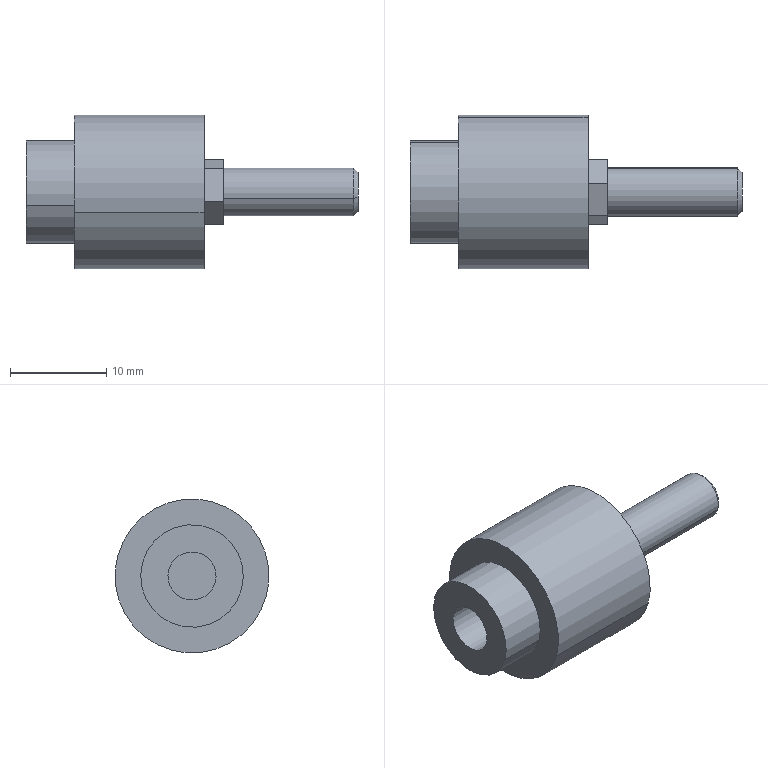Component | SolidWorks | JA15_5_080-2 | 1 solid | 22 faces | box 34.5 x 16 x 16 mm | volume 3290 mm3 | plane 12 | cylinder 8 | cone 2 | commonest cylinder face diameters 5 x4 10.667 x2 16 x2 | material 45
STEP:
#1=COLOUR_RGB('',0.7922,0.8196,0.9333);
#2=FILL_AREA_STYLE_COLOUR('',#1);
#3=FILL_AREA_STYLE('',(#2));
#4=SURFACE_STYLE_FILL_AREA(#3);
#5=SURFACE_SIDE_STYLE('',(#4));
#6=SURFACE_STYLE_USAGE(.BOTH.,#5);
#7=PRESENTATION_STYLE_ASSIGNMENT((#6));
#8=CARTESIAN_POINT('',(4.538,0.8016,3.156));
#9=VERTEX_POINT('',#8);
#10=CARTESIAN_POINT('',(4.538,0.9912,3.209));
#11=VERTEX_POINT('',#10);
#12=CARTESIAN_POINT('',(4.538,0.8964,3.182));
#13=DIRECTION('',(-1.,-0.,-0.));
#14=DIRECTION('',(0.,0.9628,0.2701));
#15=AXIS2_PLACEMENT_3D('',#12,#13,#14);
#16=CIRCLE('',#15,0.09843);
#17=EDGE_CURVE('',#9,#11,#16,.T.);
#18=ORIENTED_EDGE('',*,*,#17,.T.);
#19=CARTESIAN_POINT('',(4.952,0.9912,3.209));
#20=VERTEX_POINT('',#19);
#21=CARTESIAN_POINT('',(4.125,0.9912,3.209));
#22=DIRECTION('',(1.,0.,0.));
#23=VECTOR('',#22,39.37);
#24=LINE('',#21,#23);
#25=EDGE_CURVE('',#11,#20,#24,.T.);
#26=ORIENTED_EDGE('',*,*,#25,.T.);
#27=CARTESIAN_POINT('',(4.952,0.8016,3.156));
#28=VERTEX_POINT('',#27);
#29=CARTESIAN_POINT('',(4.952,0.8964,3.182));
#30=DIRECTION('',(1.,0.,0.));
#31=DIRECTION('',(0.,-0.9628,-0.2701));
#32=AXIS2_PLACEMENT_3D('',#29,#30,#31);
#33=CIRCLE('',#32,0.09843);
#34=EDGE_CURVE('',#20,#28,#33,.T.);
#35=ORIENTED_EDGE('',*,*,#34,.T.);
#36=CARTESIAN_POINT('',(4.125,0.8016,3.156));
#37=DIRECTION('',(1.,0.,0.));
#38=VECTOR('',#37,39.37);
#39=LINE('',#36,#38);
#40=EDGE_CURVE('',#9,#28,#39,.T.);
#41=ORIENTED_EDGE('',*,*,#40,.F.);
#42=EDGE_LOOP('',(#18,#26,#35,#41));
#43=FACE_OUTER_BOUND('',#42,.T.);
#44=CARTESIAN_POINT('',(4.125,0.8964,3.182));
#45=DIRECTION('',(1.,0.,0.));
#46=DIRECTION('',(0.,-0.9628,-0.2701));
#47=AXIS2_PLACEMENT_3D('',#44,#45,#46);
#48=CYLINDRICAL_SURFACE('',#47,0.09843);
#49=ADVANCED_FACE('',(#43),#48,.F.);
#50=CARTESIAN_POINT('',(5.877,0.9912,3.209));
#51=VERTEX_POINT('',#50);
#52=CARTESIAN_POINT('',(5.877,0.8016,3.156));
#53=VERTEX_POINT('',#52);
#54=CARTESIAN_POINT('',(5.877,0.8964,3.182));
#55=DIRECTION('',(-1.,-0.,-0.));
#56=DIRECTION('',(0.,0.9628,0.2701));
#57=AXIS2_PLACEMENT_3D('',#54,#55,#56);
#58=CIRCLE('',#57,0.09843);
#59=EDGE_CURVE('',#51,#53,#58,.T.);
#60=ORIENTED_EDGE('',*,*,#59,.T.);
#61=CARTESIAN_POINT('',(5.345,0.8016,3.156));
#62=VERTEX_POINT('',#61);
#63=CARTESIAN_POINT('',(5.345,0.8016,3.156));
#64=DIRECTION('',(-1.,-0.,-0.));
#65=VECTOR('',#64,39.37);
#66=LINE('',#63,#65);
#67=EDGE_CURVE('',#53,#62,#66,.T.);
#68=ORIENTED_EDGE('',*,*,#67,.T.);
#69=CARTESIAN_POINT('',(5.345,0.9912,3.209));
#70=VERTEX_POINT('',#69);
#71=CARTESIAN_POINT('',(5.345,0.8964,3.182));
#72=DIRECTION('',(1.,0.,0.));
#73=DIRECTION('',(0.,-0.9628,-0.2701));
#74=AXIS2_PLACEMENT_3D('',#71,#72,#73);
#75=CIRCLE('',#74,0.09843);
#76=EDGE_CURVE('',#62,#70,#75,.T.);
#77=ORIENTED_EDGE('',*,*,#76,.T.);
#78=CARTESIAN_POINT('',(5.345,0.9912,3.209));
#79=DIRECTION('',(-1.,-0.,-0.));
#80=VECTOR('',#79,39.37);
#81=LINE('',#78,#80);
#82=EDGE_CURVE('',#51,#70,#81,.T.);
#83=ORIENTED_EDGE('',*,*,#82,.F.);
#84=EDGE_LOOP('',(#60,#68,#77,#83));
#85=FACE_OUTER_BOUND('',#84,.T.);
#86=CARTESIAN_POINT('',(5.345,0.8964,3.182));
#87=DIRECTION('',(-1.,-0.,-0.));
#88=DIRECTION('',(0.,0.9628,0.2701));
#89=AXIS2_PLACEMENT_3D('',#86,#87,#88);
#90=CYLINDRICAL_SURFACE('',#89,0.09843);
#91=ADVANCED_FACE('',(#85),#90,.T.);
#92=CARTESIAN_POINT('',(5.896,0.9726,3.204));
#93=VERTEX_POINT('',#92);
#94=CARTESIAN_POINT('',(5.896,0.8202,3.161));
#95=VERTEX_POINT('',#94);
#96=CARTESIAN_POINT('',(5.896,0.8964,3.182));
#97=DIRECTION('',(-1.,-0.,-0.));
#98=DIRECTION('',(0.,0.9628,0.2701));
#99=AXIS2_PLACEMENT_3D('',#96,#97,#98);
#100=CIRCLE('',#99,0.07913);
#101=EDGE_CURVE('',#93,#95,#100,.T.);
#102=ORIENTED_EDGE('',*,*,#101,.T.);
#103=CARTESIAN_POINT('',(5.877,0.8016,3.156));
#104=DIRECTION('',(-0.7071,-0.6808,-0.191));
#105=VECTOR('',#104,39.37);
#106=LINE('',#103,#105);
#107=EDGE_CURVE('',#95,#53,#106,.T.);
#108=ORIENTED_EDGE('',*,*,#107,.T.);
#109=ORIENTED_EDGE('',*,*,#59,.F.);
#110=CARTESIAN_POINT('',(5.877,0.9912,3.209));
#111=DIRECTION('',(-0.7071,0.6808,0.191));
#112=VECTOR('',#111,39.37);
#113=LINE('',#110,#112);
#114=EDGE_CURVE('',#93,#51,#113,.T.);
#115=ORIENTED_EDGE('',*,*,#114,.F.);
#116=EDGE_LOOP('',(#102,#108,#109,#115));
#117=FACE_OUTER_BOUND('',#116,.T.);
#118=CARTESIAN_POINT('',(5.877,0.8964,3.182));
#119=DIRECTION('',(-1.,-0.,-0.));
#120=DIRECTION('',(0.,0.9628,0.2701));
#121=AXIS2_PLACEMENT_3D('',#118,#119,#120);
#122=CONICAL_SURFACE('',#121,0.09843,0.7854);
#123=ADVANCED_FACE('',(#117),#122,.T.);
#124=CARTESIAN_POINT('',(4.735,1.099,3.239));
#125=VERTEX_POINT('',#124);
#126=CARTESIAN_POINT('',(4.735,0.6942,3.126));
#127=VERTEX_POINT('',#126);
#128=CARTESIAN_POINT('',(4.735,0.8964,3.182));
#129=DIRECTION('',(-1.,-0.,-0.));
#130=DIRECTION('',(0.,0.9628,0.2701));
#131=AXIS2_PLACEMENT_3D('',#128,#129,#130);
#132=CIRCLE('',#131,0.21);
#133=EDGE_CURVE('',#125,#127,#132,.T.);
#134=ORIENTED_EDGE('',*,*,#133,.T.);
#135=CARTESIAN_POINT('',(4.538,0.6942,3.126));
#136=VERTEX_POINT('',#135);
#137=CARTESIAN_POINT('',(4.538,0.6942,3.126));
#138=DIRECTION('',(-1.,-0.,-0.));
#139=VECTOR('',#138,39.37);
#140=LINE('',#137,#139);
#141=EDGE_CURVE('',#127,#136,#140,.T.);
#142=ORIENTED_EDGE('',*,*,#141,.T.);
#143=CARTESIAN_POINT('',(4.538,1.099,3.239));
#144=VERTEX_POINT('',#143);
#145=CARTESIAN_POINT('',(4.538,0.8964,3.182));
#146=DIRECTION('',(-1.,-0.,-0.));
#147=DIRECTION('',(0.,0.9628,0.2701));
#148=AXIS2_PLACEMENT_3D('',#145,#146,#147);
#149=CIRCLE('',#148,0.21);
#150=EDGE_CURVE('',#144,#136,#149,.T.);
#151=ORIENTED_EDGE('',*,*,#150,.F.);
#152=CARTESIAN_POINT('',(4.538,1.099,3.239));
#153=DIRECTION('',(-1.,-0.,-0.));
#154=VECTOR('',#153,39.37);
#155=LINE('',#152,#154);
#156=EDGE_CURVE('',#125,#144,#155,.T.);
#157=ORIENTED_EDGE('',*,*,#156,.F.);
#158=EDGE_LOOP('',(#134,#142,#151,#157));
#159=FACE_OUTER_BOUND('',#158,.T.);
#160=CARTESIAN_POINT('',(4.538,0.8964,3.182));
#161=DIRECTION('',(-1.,-0.,-0.));
#162=DIRECTION('',(0.,0.9628,0.2701));
#163=AXIS2_PLACEMENT_3D('',#160,#161,#162);
#164=CYLINDRICAL_SURFACE('',#163,0.21);
#165=ADVANCED_FACE('',(#159),#164,.T.);
#166=CARTESIAN_POINT('',(5.267,1.2,3.267));
#167=VERTEX_POINT('',#166);
#168=CARTESIAN_POINT('',(5.267,0.5931,3.097));
#169=VERTEX_POINT('',#168);
#170=CARTESIAN_POINT('',(5.267,0.8964,3.182));
#171=DIRECTION('',(-1.,-0.,-0.));
#172=DIRECTION('',(0.,0.9628,0.2701));
#173=AXIS2_PLACEMENT_3D('',#170,#171,#172);
#174=CIRCLE('',#173,0.315);
#175=EDGE_CURVE('',#167,#169,#174,.T.);
#176=ORIENTED_EDGE('',*,*,#175,.T.);
#177=CARTESIAN_POINT('',(4.735,0.5931,3.097));
#178=VERTEX_POINT('',#177);
#179=CARTESIAN_POINT('',(4.538,0.5931,3.097));
#180=DIRECTION('',(-1.,-0.,-0.));
#181=VECTOR('',#180,39.37);
#182=LINE('',#179,#181);
#183=EDGE_CURVE('',#169,#178,#182,.T.);
#184=ORIENTED_EDGE('',*,*,#183,.T.);
#185=CARTESIAN_POINT('',(4.735,1.2,3.267));
#186=VERTEX_POINT('',#185);
#187=CARTESIAN_POINT('',(4.735,0.8964,3.182));
#188=DIRECTION('',(-1.,-0.,-0.));
#189=DIRECTION('',(0.,0.9628,0.2701));
#190=AXIS2_PLACEMENT_3D('',#187,#188,#189);
#191=CIRCLE('',#190,0.315);
#192=EDGE_CURVE('',#186,#178,#191,.T.);
#193=ORIENTED_EDGE('',*,*,#192,.F.);
#194=CARTESIAN_POINT('',(4.538,1.2,3.267));
#195=DIRECTION('',(-1.,-0.,-0.));
#196=VECTOR('',#195,39.37);
#197=LINE('',#194,#196);
#198=EDGE_CURVE('',#167,#186,#197,.T.);
#199=ORIENTED_EDGE('',*,*,#198,.F.);
#200=EDGE_LOOP('',(#176,#184,#193,#199));
#201=FACE_OUTER_BOUND('',#200,.T.);
#202=CARTESIAN_POINT('',(4.538,0.8964,3.182));
#203=DIRECTION('',(-1.,-0.,-0.));
#204=DIRECTION('',(0.,0.9628,0.2701));
#205=AXIS2_PLACEMENT_3D('',#202,#203,#204);
#206=CYLINDRICAL_SURFACE('',#205,0.315);
#207=ADVANCED_FACE('',(#201),#206,.T.);
#208=ORIENTED_EDGE('',*,*,#175,.F.);
#209=CARTESIAN_POINT('',(5.267,0.8964,3.182));
#210=DIRECTION('',(-1.,-0.,-0.));
#211=DIRECTION('',(0.,0.9628,0.2701));
#212=AXIS2_PLACEMENT_3D('',#209,#210,#211);
#213=CIRCLE('',#212,0.315);
#214=EDGE_CURVE('',#169,#167,#213,.T.);
#215=ORIENTED_EDGE('',*,*,#214,.F.);
#216=EDGE_LOOP('',(#208,#215));
#217=FACE_OUTER_BOUND('',#216,.T.);
#218=CARTESIAN_POINT('',(5.267,0.9301,3.314));
#219=VERTEX_POINT('',#218);
#220=CARTESIAN_POINT('',(5.267,0.7988,3.278));
#221=VERTEX_POINT('',#220);
#222=CARTESIAN_POINT('',(5.267,0.9301,3.314));
#223=DIRECTION('',(0.,-0.9628,-0.2701));
#224=VECTOR('',#223,39.37);
#225=LINE('',#222,#224);
#226=EDGE_CURVE('',#219,#221,#225,.T.);
#227=ORIENTED_EDGE('',*,*,#226,.F.);
#228=CARTESIAN_POINT('',(5.267,1.028,3.219));
#229=VERTEX_POINT('',#228);
#230=CARTESIAN_POINT('',(5.267,1.028,3.219));
#231=DIRECTION('',(-0.,-0.7154,0.6988));
#232=VECTOR('',#231,39.37);
#233=LINE('',#230,#232);
#234=EDGE_CURVE('',#229,#219,#233,.T.);
#235=ORIENTED_EDGE('',*,*,#234,.F.);
#236=CARTESIAN_POINT('',(5.267,0.994,3.087));
#237=VERTEX_POINT('',#236);
#238=CARTESIAN_POINT('',(5.267,0.994,3.087));
#239=DIRECTION('',(-0.,0.2475,0.9689));
#240=VECTOR('',#239,39.37);
#241=LINE('',#238,#240);
#242=EDGE_CURVE('',#237,#229,#241,.T.);
#243=ORIENTED_EDGE('',*,*,#242,.F.);
#244=CARTESIAN_POINT('',(5.267,0.8626,3.05));
#245=VERTEX_POINT('',#244);
#246=CARTESIAN_POINT('',(5.267,0.8626,3.05));
#247=DIRECTION('',(-0.,0.9628,0.2701));
#248=VECTOR('',#247,39.37);
#249=LINE('',#246,#248);
#250=EDGE_CURVE('',#245,#237,#249,.T.);
#251=ORIENTED_EDGE('',*,*,#250,.F.);
#252=CARTESIAN_POINT('',(5.267,0.7651,3.145));
#253=VERTEX_POINT('',#252);
#254=CARTESIAN_POINT('',(5.267,0.7651,3.145));
#255=DIRECTION('',(0.,0.7154,-0.6988));
#256=VECTOR('',#255,39.37);
#257=LINE('',#254,#256);
#258=EDGE_CURVE('',#253,#245,#257,.T.);
#259=ORIENTED_EDGE('',*,*,#258,.F.);
#260=CARTESIAN_POINT('',(5.267,0.7988,3.278));
#261=DIRECTION('',(0.,-0.2475,-0.9689));
#262=VECTOR('',#261,39.37);
#263=LINE('',#260,#262);
#264=EDGE_CURVE('',#221,#253,#263,.T.);
#265=ORIENTED_EDGE('',*,*,#264,.F.);
#266=EDGE_LOOP('',(#227,#235,#243,#251,#259,#265));
#267=FACE_BOUND('',#266,.T.);
#268=CARTESIAN_POINT('',(5.267,0.8964,3.182));
#269=DIRECTION('',(1.,0.,0.));
#270=DIRECTION('',(0.,-0.9628,-0.2701));
#271=AXIS2_PLACEMENT_3D('',#268,#269,#270);
#272=PLANE('',#271);
#273=ADVANCED_FACE('',(#217,#267),#272,.T.);
#274=ORIENTED_EDGE('',*,*,#183,.F.);
#275=ORIENTED_EDGE('',*,*,#214,.T.);
#276=ORIENTED_EDGE('',*,*,#198,.T.);
#277=CARTESIAN_POINT('',(4.735,0.8964,3.182));
#278=DIRECTION('',(-1.,-0.,-0.));
#279=DIRECTION('',(0.,0.9628,0.2701));
#280=AXIS2_PLACEMENT_3D('',#277,#278,#279);
#281=CIRCLE('',#280,0.315);
#282=EDGE_CURVE('',#178,#186,#281,.T.);
#283=ORIENTED_EDGE('',*,*,#282,.F.);
#284=EDGE_LOOP('',(#274,#275,#276,#283));
#285=FACE_OUTER_BOUND('',#284,.T.);
#286=CARTESIAN_POINT('',(4.538,0.8964,3.182));
#287=DIRECTION('',(-1.,-0.,-0.));
#288=DIRECTION('',(0.,0.9628,0.2701));
#289=AXIS2_PLACEMENT_3D('',#286,#287,#288);
#290=CYLINDRICAL_SURFACE('',#289,0.315);
#291=ADVANCED_FACE('',(#285),#290,.T.);
#292=ORIENTED_EDGE('',*,*,#192,.T.);
#293=ORIENTED_EDGE('',*,*,#282,.T.);
#294=EDGE_LOOP('',(#292,#293));
#295=FACE_OUTER_BOUND('',#294,.T.);
#296=ORIENTED_EDGE('',*,*,#133,.F.);
#297=CARTESIAN_POINT('',(4.735,0.8964,3.182));
#298=DIRECTION('',(-1.,-0.,-0.));
#299=DIRECTION('',(0.,0.9628,0.2701));
#300=AXIS2_PLACEMENT_3D('',#297,#298,#299);
#301=CIRCLE('',#300,0.21);
#302=EDGE_CURVE('',#127,#125,#301,.T.);
#303=ORIENTED_EDGE('',*,*,#302,.F.);
#304=EDGE_LOOP('',(#296,#303));
#305=FACE_BOUND('',#304,.T.);
#306=CARTESIAN_POINT('',(4.735,0.9815,2.879));
#307=DIRECTION('',(-1.,-0.,-0.));
#308=DIRECTION('',(-0.,0.9628,0.2701));
#309=AXIS2_PLACEMENT_3D('',#306,#307,#308);
#310=PLANE('',#309);
#311=ADVANCED_FACE('',(#295,#305),#310,.T.);
#312=ORIENTED_EDGE('',*,*,#141,.F.);
#313=ORIENTED_EDGE('',*,*,#302,.T.);
#314=ORIENTED_EDGE('',*,*,#156,.T.);
#315=CARTESIAN_POINT('',(4.538,0.8964,3.182));
#316=DIRECTION('',(-1.,-0.,-0.));
#317=DIRECTION('',(0.,0.9628,0.2701));
#318=AXIS2_PLACEMENT_3D('',#315,#316,#317);
#319=CIRCLE('',#318,0.21);
#320=EDGE_CURVE('',#136,#144,#319,.T.);
#321=ORIENTED_EDGE('',*,*,#320,.F.);
#322=EDGE_LOOP('',(#312,#313,#314,#321));
#323=FACE_OUTER_BOUND('',#322,.T.);
#324=CARTESIAN_POINT('',(4.538,0.8964,3.182));
#325=DIRECTION('',(-1.,-0.,-0.));
#326=DIRECTION('',(0.,0.9628,0.2701));
#327=AXIS2_PLACEMENT_3D('',#324,#325,#326);
#328=CYLINDRICAL_SURFACE('',#327,0.21);
#329=ADVANCED_FACE('',(#323),#328,.T.);
#330=ORIENTED_EDGE('',*,*,#150,.T.);
#331=ORIENTED_EDGE('',*,*,#320,.T.);
#332=EDGE_LOOP('',(#330,#331));
#333=FACE_OUTER_BOUND('',#332,.T.);
#334=ORIENTED_EDGE('',*,*,#17,.F.);
#335=CARTESIAN_POINT('',(4.538,0.8964,3.182));
#336=DIRECTION('',(-1.,-0.,-0.));
#337=DIRECTION('',(0.,0.9628,0.2701));
#338=AXIS2_PLACEMENT_3D('',#335,#336,#337);
#339=CIRCLE('',#338,0.09843);
#340=EDGE_CURVE('',#11,#9,#339,.T.);
#341=ORIENTED_EDGE('',*,*,#340,.F.);
#342=EDGE_LOOP('',(#334,#341));
#343=FACE_BOUND('',#342,.T.);
#344=CARTESIAN_POINT('',(4.538,0.9531,2.98));
#345=DIRECTION('',(-1.,-0.,-0.));
#346=DIRECTION('',(-0.,0.9628,0.2701));
#347=AXIS2_PLACEMENT_3D('',#344,#345,#346);
#348=PLANE('',#347);
#349=ADVANCED_FACE('',(#333,#343),#348,.T.);
#350=ORIENTED_EDGE('',*,*,#234,.T.);
#351=CARTESIAN_POINT('',(5.345,0.9301,3.314));
#352=VERTEX_POINT('',#351);
#353=CARTESIAN_POINT('',(5.345,0.9301,3.314));
#354=DIRECTION('',(-1.,-0.,-0.));
#355=VECTOR('',#354,39.37);
#356=LINE('',#353,#355);
#357=EDGE_CURVE('',#352,#219,#356,.T.);
#358=ORIENTED_EDGE('',*,*,#357,.F.);
#359=CARTESIAN_POINT('',(5.345,1.028,3.219));
#360=VERTEX_POINT('',#359);
#361=CARTESIAN_POINT('',(5.345,1.028,3.219));
#362=DIRECTION('',(-0.,-0.7154,0.6988));
#363=VECTOR('',#362,39.37);
#364=LINE('',#361,#363);
#365=EDGE_CURVE('',#360,#352,#364,.T.);
#366=ORIENTED_EDGE('',*,*,#365,.F.);
#367=CARTESIAN_POINT('',(5.345,1.028,3.219));
#368=DIRECTION('',(-1.,-0.,-0.));
#369=VECTOR('',#368,39.37);
#370=LINE('',#367,#369);
#371=EDGE_CURVE('',#360,#229,#370,.T.);
#372=ORIENTED_EDGE('',*,*,#371,.T.);
#373=EDGE_LOOP('',(#350,#358,#366,#372));
#374=FACE_OUTER_BOUND('',#373,.T.);
#375=CARTESIAN_POINT('',(5.345,1.028,3.219));
#376=DIRECTION('',(0.,-0.6988,-0.7154));
#377=DIRECTION('',(0.,0.7154,-0.6988));
#378=AXIS2_PLACEMENT_3D('',#375,#376,#377);
#379=PLANE('',#378);
#380=ADVANCED_FACE('',(#374),#379,.F.);
#381=ORIENTED_EDGE('',*,*,#226,.T.);
#382=CARTESIAN_POINT('',(5.345,0.7988,3.278));
#383=VERTEX_POINT('',#382);
#384=CARTESIAN_POINT('',(5.345,0.7988,3.278));
#385=DIRECTION('',(-1.,-0.,-0.));
#386=VECTOR('',#385,39.37);
#387=LINE('',#384,#386);
#388=EDGE_CURVE('',#383,#221,#387,.T.);
#389=ORIENTED_EDGE('',*,*,#388,.F.);
#390=CARTESIAN_POINT('',(5.345,0.9301,3.314));
#391=DIRECTION('',(0.,-0.9628,-0.2701));
#392=VECTOR('',#391,39.37);
#393=LINE('',#390,#392);
#394=EDGE_CURVE('',#352,#383,#393,.T.);
#395=ORIENTED_EDGE('',*,*,#394,.F.);
#396=ORIENTED_EDGE('',*,*,#357,.T.);
#397=EDGE_LOOP('',(#381,#389,#395,#396));
#398=FACE_OUTER_BOUND('',#397,.T.);
#399=CARTESIAN_POINT('',(5.345,0.9301,3.314));
#400=DIRECTION('',(0.,0.2701,-0.9628));
#401=DIRECTION('',(1.,0.,0.));
#402=AXIS2_PLACEMENT_3D('',#399,#400,#401);
#403=PLANE('',#402);
#404=ADVANCED_FACE('',(#398),#403,.F.);
#405=ORIENTED_EDGE('',*,*,#264,.T.);
#406=CARTESIAN_POINT('',(5.345,0.7651,3.145));
#407=VERTEX_POINT('',#406);
#408=CARTESIAN_POINT('',(5.345,0.7651,3.145));
#409=DIRECTION('',(-1.,-0.,-0.));
#410=VECTOR('',#409,39.37);
#411=LINE('',#408,#410);
#412=EDGE_CURVE('',#407,#253,#411,.T.);
#413=ORIENTED_EDGE('',*,*,#412,.F.);
#414=CARTESIAN_POINT('',(5.345,0.7988,3.278));
#415=DIRECTION('',(0.,-0.2475,-0.9689));
#416=VECTOR('',#415,39.37);
#417=LINE('',#414,#416);
#418=EDGE_CURVE('',#383,#407,#417,.T.);
#419=ORIENTED_EDGE('',*,*,#418,.F.);
#420=ORIENTED_EDGE('',*,*,#388,.T.);
#421=EDGE_LOOP('',(#405,#413,#419,#420));
#422=FACE_OUTER_BOUND('',#421,.T.);
#423=CARTESIAN_POINT('',(5.345,0.7988,3.278));
#424=DIRECTION('',(0.,0.9689,-0.2475));
#425=DIRECTION('',(-0.,0.2475,0.9689));
#426=AXIS2_PLACEMENT_3D('',#423,#424,#425);
#427=PLANE('',#426);
#428=ADVANCED_FACE('',(#422),#427,.F.);
#429=ORIENTED_EDGE('',*,*,#258,.T.);
#430=CARTESIAN_POINT('',(5.345,0.8626,3.05));
#431=VERTEX_POINT('',#430);
#432=CARTESIAN_POINT('',(5.345,0.8626,3.05));
#433=DIRECTION('',(-1.,-0.,-0.));
#434=VECTOR('',#433,39.37);
#435=LINE('',#432,#434);
#436=EDGE_CURVE('',#431,#245,#435,.T.);
#437=ORIENTED_EDGE('',*,*,#436,.F.);
#438=CARTESIAN_POINT('',(5.345,0.7651,3.145));
#439=DIRECTION('',(0.,0.7154,-0.6988));
#440=VECTOR('',#439,39.37);
#441=LINE('',#438,#440);
#442=EDGE_CURVE('',#407,#431,#441,.T.);
#443=ORIENTED_EDGE('',*,*,#442,.F.);
#444=ORIENTED_EDGE('',*,*,#412,.T.);
#445=EDGE_LOOP('',(#429,#437,#443,#444));
#446=FACE_OUTER_BOUND('',#445,.T.);
#447=CARTESIAN_POINT('',(5.345,0.7651,3.145));
#448=DIRECTION('',(-0.,0.6988,0.7154));
#449=DIRECTION('',(-0.,-0.7154,0.6988));
#450=AXIS2_PLACEMENT_3D('',#447,#448,#449);
#451=PLANE('',#450);
#452=ADVANCED_FACE('',(#446),#451,.F.);
#453=ORIENTED_EDGE('',*,*,#250,.T.);
#454=CARTESIAN_POINT('',(5.345,0.994,3.087));
#455=VERTEX_POINT('',#454);
#456=CARTESIAN_POINT('',(5.345,0.994,3.087));
#457=DIRECTION('',(-1.,-0.,-0.));
#458=VECTOR('',#457,39.37);
#459=LINE('',#456,#458);
#460=EDGE_CURVE('',#455,#237,#459,.T.);
#461=ORIENTED_EDGE('',*,*,#460,.F.);
#462=CARTESIAN_POINT('',(5.345,0.8626,3.05));
#463=DIRECTION('',(-0.,0.9628,0.2701));
#464=VECTOR('',#463,39.37);
#465=LINE('',#462,#464);
#466=EDGE_CURVE('',#431,#455,#465,.T.);
#467=ORIENTED_EDGE('',*,*,#466,.F.);
#468=ORIENTED_EDGE('',*,*,#436,.T.);
#469=EDGE_LOOP('',(#453,#461,#467,#468));
#470=FACE_OUTER_BOUND('',#469,.T.);
#471=CARTESIAN_POINT('',(5.345,0.8626,3.05));
#472=DIRECTION('',(-0.,-0.2701,0.9628));
#473=DIRECTION('',(-1.,-0.,-0.));
#474=AXIS2_PLACEMENT_3D('',#471,#472,#473);
#475=PLANE('',#474);
#476=ADVANCED_FACE('',(#470),#475,.F.);
#477=ORIENTED_EDGE('',*,*,#242,.T.);
#478=ORIENTED_EDGE('',*,*,#371,.F.);
#479=CARTESIAN_POINT('',(5.345,0.994,3.087));
#480=DIRECTION('',(-0.,0.2475,0.9689));
#481=VECTOR('',#480,39.37);
#482=LINE('',#479,#481);
#483=EDGE_CURVE('',#455,#360,#482,.T.);
#484=ORIENTED_EDGE('',*,*,#483,.F.);
#485=ORIENTED_EDGE('',*,*,#460,.T.);
#486=EDGE_LOOP('',(#477,#478,#484,#485));
#487=FACE_OUTER_BOUND('',#486,.T.);
#488=CARTESIAN_POINT('',(5.345,0.994,3.087));
#489=DIRECTION('',(-0.,-0.9689,0.2475));
#490=DIRECTION('',(0.,-0.2475,-0.9689));
#491=AXIS2_PLACEMENT_3D('',#488,#489,#490);
#492=PLANE('',#491);
#493=ADVANCED_FACE('',(#487),#492,.F.);
#494=CARTESIAN_POINT('',(5.345,0.8964,3.182));
#495=DIRECTION('',(1.,0.,0.));
#496=DIRECTION('',(0.,-0.9628,-0.2701));
#497=AXIS2_PLACEMENT_3D('',#494,#495,#496);
#498=CIRCLE('',#497,0.09843);
#499=EDGE_CURVE('',#70,#62,#498,.T.);
#500=ORIENTED_EDGE('',*,*,#499,.F.);
#501=ORIENTED_EDGE('',*,*,#76,.F.);
#502=EDGE_LOOP('',(#500,#501));
#503=FACE_BOUND('',#502,.T.);
#504=ORIENTED_EDGE('',*,*,#365,.T.);
#505=ORIENTED_EDGE('',*,*,#394,.T.);
#506=ORIENTED_EDGE('',*,*,#418,.T.);
#507=ORIENTED_EDGE('',*,*,#442,.T.);
#508=ORIENTED_EDGE('',*,*,#466,.T.);
#509=ORIENTED_EDGE('',*,*,#483,.T.);
#510=EDGE_LOOP('',(#504,#505,#506,#507,#508,#509));
#511=FACE_OUTER_BOUND('',#510,.T.);
#512=CARTESIAN_POINT('',(5.345,0.9301,3.314));
#513=DIRECTION('',(1.,0.,0.));
#514=DIRECTION('',(0.,-0.9628,-0.2701));
#515=AXIS2_PLACEMENT_3D('',#512,#513,#514);
#516=PLANE('',#515);
#517=ADVANCED_FACE('',(#503,#511),#516,.T.);
#518=ORIENTED_EDGE('',*,*,#101,.F.);
#519=CARTESIAN_POINT('',(5.896,0.8964,3.182));
#520=DIRECTION('',(-1.,-0.,-0.));
#521=DIRECTION('',(0.,0.9628,0.2701));
#522=AXIS2_PLACEMENT_3D('',#519,#520,#521);
#523=CIRCLE('',#522,0.07913);
#524=EDGE_CURVE('',#95,#93,#523,.T.);
#525=ORIENTED_EDGE('',*,*,#524,.F.);
#526=EDGE_LOOP('',(#518,#525));
#527=FACE_OUTER_BOUND('',#526,.T.);
#528=CARTESIAN_POINT('',(5.896,0.8964,3.182));
#529=DIRECTION('',(1.,0.,0.));
#530=DIRECTION('',(0.,-0.9628,-0.2701));
#531=AXIS2_PLACEMENT_3D('',#528,#529,#530);
#532=PLANE('',#531);
#533=ADVANCED_FACE('',(#527),#532,.T.);
#534=ORIENTED_EDGE('',*,*,#107,.F.);
#535=ORIENTED_EDGE('',*,*,#524,.T.);
#536=ORIENTED_EDGE('',*,*,#114,.T.);
#537=CARTESIAN_POINT('',(5.877,0.8964,3.182));
#538=DIRECTION('',(-1.,-0.,-0.));
#539=DIRECTION('',(0.,0.9628,0.2701));
#540=AXIS2_PLACEMENT_3D('',#537,#538,#539);
#541=CIRCLE('',#540,0.09843);
#542=EDGE_CURVE('',#53,#51,#541,.T.);
#543=ORIENTED_EDGE('',*,*,#542,.F.);
#544=EDGE_LOOP('',(#534,#535,#536,#543));
#545=FACE_OUTER_BOUND('',#544,.T.);
#546=CARTESIAN_POINT('',(5.877,0.8964,3.182));
#547=DIRECTION('',(-1.,-0.,-0.));
#548=DIRECTION('',(0.,0.9628,0.2701));
#549=AXIS2_PLACEMENT_3D('',#546,#547,#548);
#550=CONICAL_SURFACE('',#549,0.09843,0.7854);
#551=ADVANCED_FACE('',(#545),#550,.T.);
#552=ORIENTED_EDGE('',*,*,#67,.F.);
#553=ORIENTED_EDGE('',*,*,#542,.T.);
#554=ORIENTED_EDGE('',*,*,#82,.T.);
#555=ORIENTED_EDGE('',*,*,#499,.T.);
#556=EDGE_LOOP('',(#552,#553,#554,#555));
#557=FACE_OUTER_BOUND('',#556,.T.);
#558=CARTESIAN_POINT('',(5.345,0.8964,3.182));
#559=DIRECTION('',(-1.,-0.,-0.));
#560=DIRECTION('',(0.,0.9628,0.2701));
#561=AXIS2_PLACEMENT_3D('',#558,#559,#560);
#562=CYLINDRICAL_SURFACE('',#561,0.09843);
#563=ADVANCED_FACE('',(#557),#562,.T.);
#564=ORIENTED_EDGE('',*,*,#25,.F.);
#565=ORIENTED_EDGE('',*,*,#340,.T.);
#566=ORIENTED_EDGE('',*,*,#40,.T.);
#567=CARTESIAN_POINT('',(4.952,0.8964,3.182));
#568=DIRECTION('',(1.,0.,0.));
#569=DIRECTION('',(0.,-0.9628,-0.2701));
#570=AXIS2_PLACEMENT_3D('',#567,#568,#569);
#571=CIRCLE('',#570,0.09843);
#572=EDGE_CURVE('',#28,#20,#571,.T.);
#573=ORIENTED_EDGE('',*,*,#572,.T.);
#574=EDGE_LOOP('',(#564,#565,#566,#573));
#575=FACE_OUTER_BOUND('',#574,.T.);
#576=CARTESIAN_POINT('',(4.125,0.8964,3.182));
#577=DIRECTION('',(1.,0.,0.));
#578=DIRECTION('',(0.,-0.9628,-0.2701));
#579=AXIS2_PLACEMENT_3D('',#576,#577,#578);
#580=CYLINDRICAL_SURFACE('',#579,0.09843);
#581=ADVANCED_FACE('',(#575),#580,.F.);
#582=ORIENTED_EDGE('',*,*,#572,.F.);
#583=ORIENTED_EDGE('',*,*,#34,.F.);
#584=EDGE_LOOP('',(#582,#583));
#585=FACE_OUTER_BOUND('',#584,.T.);
#586=CARTESIAN_POINT('',(4.952,0.8964,3.182));
#587=DIRECTION('',(1.,0.,0.));
#588=DIRECTION('',(0.,-0.9628,-0.2701));
#589=AXIS2_PLACEMENT_3D('',#586,#587,#588);
#590=PLANE('',#589);
#591=ADVANCED_FACE('',(#585),#590,.F.);
#592=CLOSED_SHELL('',(#49,#91,#123,#165,#207,#273,#291,#311,#329,#349,#380,#404,#428,#452,#476,#493,#517,#533,#551,#563,#581,#591));
#593=MANIFOLD_SOLID_BREP('',#592);
#594=STYLED_ITEM('',(#7),#593);
#595=(LENGTH_UNIT()NAMED_UNIT(*)SI_UNIT($,.METRE.));
#596=LENGTH_MEASURE_WITH_UNIT(LENGTH_MEASURE(0.0254),#595);
#597=DIMENSIONAL_EXPONENTS(1.,0.,0.,0.,0.,0.,0.);
#598=(CONVERSION_BASED_UNIT('',#596)LENGTH_UNIT()NAMED_UNIT(#597));
#599=UNCERTAINTY_MEASURE_WITH_UNIT(LENGTH_MEASURE(0.00001),#598,'','');
#600=(NAMED_UNIT(*)PLANE_ANGLE_UNIT()SI_UNIT($,.RADIAN.));
#601=(NAMED_UNIT(*)SI_UNIT($,.STERADIAN.)SOLID_ANGLE_UNIT());
#602=(GEOMETRIC_REPRESENTATION_CONTEXT(3)GLOBAL_UNCERTAINTY_ASSIGNED_CONTEXT((#599))GLOBAL_UNIT_ASSIGNED_CONTEXT((#598,#600,#601))REPRESENTATION_CONTEXT('',''));
#603=MECHANICAL_DESIGN_GEOMETRIC_PRESENTATION_REPRESENTATION('',(#594),#602);
#604=PRESENTATION_LAYER_ASSIGNMENT('','',(#594));
#605=CARTESIAN_POINT('',(0.,0.,0.));
#606=DIRECTION('',(0.,0.,1.));
#607=DIRECTION('',(1.,0.,0.));
#608=AXIS2_PLACEMENT_3D('',#605,#606,#607);
#609=(LENGTH_UNIT()NAMED_UNIT(*)SI_UNIT($,.METRE.));
#610=LENGTH_MEASURE_WITH_UNIT(LENGTH_MEASURE(0.0254),#609);
#611=DIMENSIONAL_EXPONENTS(1.,0.,0.,0.,0.,0.,0.);
#612=(CONVERSION_BASED_UNIT('',#610)LENGTH_UNIT()NAMED_UNIT(#611));
#613=UNCERTAINTY_MEASURE_WITH_UNIT(LENGTH_MEASURE(0.00001),#612,'','');
#614=(NAMED_UNIT(*)PLANE_ANGLE_UNIT()SI_UNIT($,.RADIAN.));
#615=(NAMED_UNIT(*)SI_UNIT($,.STERADIAN.)SOLID_ANGLE_UNIT());
#616=(GEOMETRIC_REPRESENTATION_CONTEXT(3)GLOBAL_UNCERTAINTY_ASSIGNED_CONTEXT((#613))GLOBAL_UNIT_ASSIGNED_CONTEXT((#612,#614,#615))REPRESENTATION_CONTEXT('',''));
#617=ADVANCED_BREP_SHAPE_REPRESENTATION('',(#593,#608),#616);